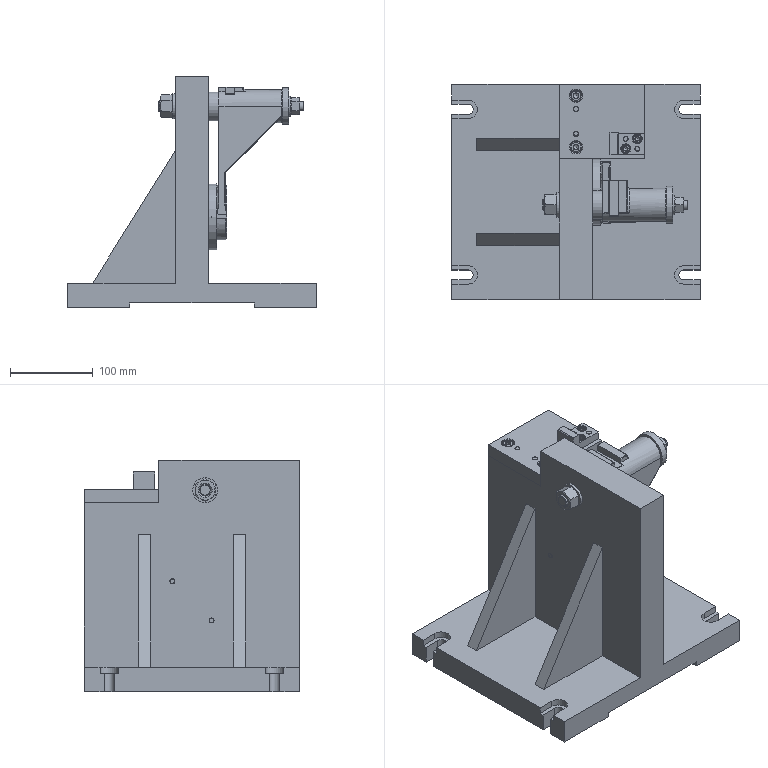Assembly | NX | mm | 25 component files | 26 solids | 560 faces | box 300 x 260 x 280 mm | volume 5149342 mm3 | plane 295 | cone 144 | cylinder 92 | torus 19 | spline 10 | commonest cylinder face diameters 6 x21 5.795 x6 10 x6 5.9 x6 6.6 x6 11 x6 13 x4 12 x4
Bill of materials:
GB-T6170_F-2000,M16x2 | 1 |  | Hexagonal nut-like body with a central through bore and chamfered corners at both faces.
GB-T70.1-2000,M8x20 | 2 |  | Hexagon Socket Head Cap Screw, GB-T 70.1-2000,M8x20
GB-T97_1-2002,M16 | 1 |  | Flat annular ring (plain washer-like disc) with a concentric circular through-hole, flat parallel faces and a plain cylindrical outer edge.
unnamed part 1 | 1 |  | Stepped cylindrical shaft or pin: a larger-diameter middle section with a smaller-diameter journal at each end.
GB-T97_1-2002,M12 | 1 |  | Flat annular ring (plain washer-like disc) with a concentric circular through-hole, flat parallel faces and a plain cylindrical outer edge. Almost identical in form to unnamed part.
unnamed part 2 | 1 |  | Flat circular disc with a straight-sided slot running from the edge to a round-ended end near the center (a C-washer or slotted-washer shape).
unnamed part 3 | 1 |  | Rectangular flat plate with two counterbored holes, two plain holes along one edge, and a cluster of four smaller holes near the opposite corner.
GB-T119.1-2000,6x50 | 2 |  | Parallel Pin, GB-T 119.1-2000,6x50
unnamed part 4 | 1 |  | L-shaped block: a thick base with an upright wall along one end, two counterbored holes and two plain holes through the base.
GB-T6170_F-2000,M12x1.75 | 1 |  | Hexagonal nut-like body with a central through bore and chamfered corners at both faces; it looks almost the same as unnamed part.
GB-T70.1-2000,M6x12 | 6 |  | Hexagon Socket Head Cap Screw, GB-T 70.1-2000,M6x12
unnamed part 5 | 1 |  | Fork-shaped arm: a cylindrical tubular hub on one end and a semicircular cutout at the other end, joined by a tapered web.
unnamed part 6 | 1 |  | Round flange or cover: a flat circular disc with a raised concentric circular spigot on one face and a ring of six holes.
GB-T119.1-2000,6x26 | 4 |  | Parallel Pin, GB-T 119.1-2000,6x26
unnamed part 7 | 1 |  | Angle bracket or stand: a rectangular base plate with an upright plate supported by a triangular gusset; the upright carries a stepped boss and small hole patterns.
Mates:
1. fix | fixture_body 1 component
2. concentric | locating_block 1 | fixture_body 1
3. touch align | locating_block 1 face | fixture_body 1 face
4. touch align | BOCHAlingjian 1 face | locating_block 1 face
5. parallel | BOCHAlingjian 1 face | fixture_body 1 face
6. touch align | BOCHAlingjian 1 face | locating_block 1 face
7. touch align | tool_setting_block 1 face | BOCHAlingjian 1 face
8. touch align | tool_setting_block 1 face | BOCHAlingjian 1 face
9. concentric | shim_block 1 edge | fixture_body 1 edge
10. touch align | shim_block 1 face | fixture_body 1 face
11. distance | tool_setting_block 1 face | fixture_body 1 face
12. concentric | threaded_rod 1 edge | fixture_body 1 edge
13. concentric | GB-T97_1-2002_M16 1 edge | fixture_body 1 edge
14. concentric | GB-T6170_F-2000_M16x2 1 edge | GB-T97_1-2002_M16 1 edge
15. concentric | split_washer 1 edge | BOCHAlingjian 1 edge
16. concentric | GB-T97_1-2002_M12 1 edge | split_washer 1 edge
17. concentric | GB-T6170_F-2000_M12x1_75 1 edge | GB-T97_1-2002_M12 1 edge
18. concentric | GB-T70_1-2000_M6x12 6 edge | locating_block 1 edge
19. bond | locating_block 1 component | assembly component
20. bond | GB-T70_1-2000_M6x12 6 component | assembly component
21. bond | GB-T70_1-2000_M6x12 5 component | assembly component
22. bond | GB-T70_1-2000_M6x12 4 component | assembly component
23. circular | assembly datumaxis | assembly cartesiancoordinatesystem | assembly cartesiancoordinatesystem | assembly cartesiancoordinatesystem | assembly cartesiancoordinatesystem
24. bond | GB-T70_1-2000_M6x12 3 component | assembly component
25. concentric | GB-T119_1-2000_6x50 2 edge | locating_block 1 edge
26. bond | locating_block 1 component | assembly component
27. bond | GB-T119_1-2000_6x50 2 component | assembly component
28. bond | GB-T119_1-2000_6x50 1 component | assembly component
29. circular | assembly datumaxis | assembly cartesiancoordinatesystem | assembly cartesiancoordinatesystem
30. concentric | GB-T70_1-2000_M6x12 2 edge | tool_setting_block 1 edge
31. concentric | GB-T70_1-2000_M6x12 1 edge | tool_setting_block 1 edge
32. concentric | GB-T119_1-2000_6x26 4 edge | tool_setting_block 1 edge
33. concentric | GB-T119_1-2000_6x26 3 edge | tool_setting_block 1 edge
34. concentric | GB-T119_1-2000_6x26 1 edge | shim_block 1 edge
35. concentric | GB-T119_1-2000_6x26 2 edge | shim_block 1 edge
36. concentric | GB-T70_1-2000_M8x20 2 edge | shim_block 1 edge
37. concentric | GB-T70_1-2000_M8x20 1 edge | shim_block 1 edge